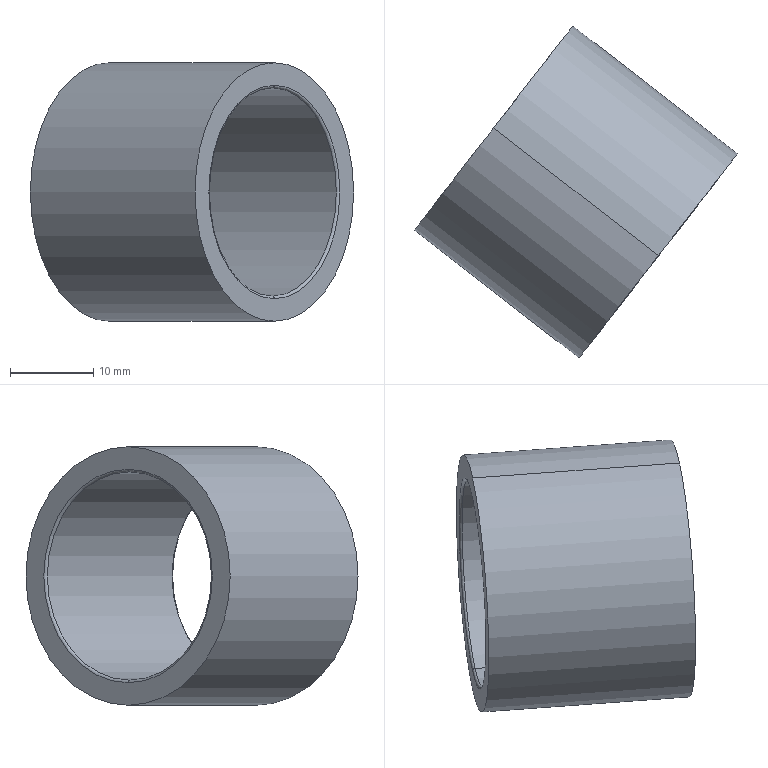Component | SolidWorks | MISUMI_BSSRK3210-800-F34-P20-1_COLLAR_MISUMI_BSSRK3210-800-F34-P20-1 | 1 solid | 10 faces | box 38.76 x 39.82 x 31 mm | volume 6594 mm3 | cylinder 4 | torus 4 | plane 2 | commonest cylinder face diameters 31 x2 25 x2
build123d program:
from build123d import *


with BuildPart() as part:
    # Sketch1 → Revolve1 (revolve)
    with BuildSketch(Plane.XY, mode=Mode.PRIVATE) as revolve1_sk:
        with BuildLine():
            Line((0.3, 12.5), (24.7, 12.5))
            ThreePointArc((24.7, 12.5), (24.912, 12.588), (25, 12.8))
            Line((25, 12.8), (25, 15.5))
            Line((25, 15.5), (0, 15.5))
            Line((0, 15.5), (0, 12.8))
            ThreePointArc((0, 12.8), (0.08787, 12.588), (0.3, 12.5))
        make_face()
    revolve(revolve1_sk.sketch.rotate(Axis((0, 0, 0), (1, 0, 0)), 90), axis=Axis((0, 0, 0), (1, 0, 0)))


solid = part.part

# Placed as in the assembly
solid = solid.moved(Location((-94.863, 818.28, 276.411), (-65.606, 35.259, -14.67)))
STEP:
#1=COLOUR_RGB('',0.7922,0.8196,0.9333);
#2=FILL_AREA_STYLE_COLOUR('',#1);
#3=FILL_AREA_STYLE('',(#2));
#4=SURFACE_STYLE_FILL_AREA(#3);
#5=SURFACE_SIDE_STYLE('',(#4));
#6=SURFACE_STYLE_USAGE(.BOTH.,#5);
#7=PRESENTATION_STYLE_ASSIGNMENT((#6));
#8=CARTESIAN_POINT('',(-3.735,32.216,11.493));
#9=VERTEX_POINT('',#8);
#10=CARTESIAN_POINT('',(-3.735,32.216,10.272));
#11=VERTEX_POINT('',#10);
#12=CARTESIAN_POINT('',(-3.735,32.216,10.882));
#13=DIRECTION('',(0.7899,-0.6132,-0.));
#14=DIRECTION('',(-0.,-0.,1.));
#15=AXIS2_PLACEMENT_3D('',#12,#13,#14);
#16=CIRCLE('',#15,0.6102);
#17=EDGE_CURVE('',#9,#11,#16,.T.);
#18=ORIENTED_EDGE('',*,*,#17,.T.);
#19=CARTESIAN_POINT('',(-2.957,31.612,10.272));
#20=VERTEX_POINT('',#19);
#21=CARTESIAN_POINT('',(-2.957,31.612,10.272));
#22=DIRECTION('',(0.7899,-0.6132,-0.));
#23=VECTOR('',#22,39.37);
#24=LINE('',#21,#23);
#25=EDGE_CURVE('',#11,#20,#24,.T.);
#26=ORIENTED_EDGE('',*,*,#25,.T.);
#27=CARTESIAN_POINT('',(-2.957,31.612,11.493));
#28=VERTEX_POINT('',#27);
#29=CARTESIAN_POINT('',(-2.957,31.612,10.882));
#30=DIRECTION('',(0.7899,-0.6132,-0.));
#31=DIRECTION('',(-0.,-0.,1.));
#32=AXIS2_PLACEMENT_3D('',#29,#30,#31);
#33=CIRCLE('',#32,0.6102);
#34=EDGE_CURVE('',#28,#20,#33,.T.);
#35=ORIENTED_EDGE('',*,*,#34,.F.);
#36=CARTESIAN_POINT('',(-2.957,31.612,11.493));
#37=DIRECTION('',(0.7899,-0.6132,-0.));
#38=VECTOR('',#37,39.37);
#39=LINE('',#36,#38);
#40=EDGE_CURVE('',#9,#28,#39,.T.);
#41=ORIENTED_EDGE('',*,*,#40,.F.);
#42=EDGE_LOOP('',(#18,#26,#35,#41));
#43=FACE_OUTER_BOUND('',#42,.T.);
#44=CARTESIAN_POINT('',(-2.957,31.612,10.882));
#45=DIRECTION('',(0.7899,-0.6132,-0.));
#46=DIRECTION('',(-0.,-0.,1.));
#47=AXIS2_PLACEMENT_3D('',#44,#45,#46);
#48=CYLINDRICAL_SURFACE('',#47,0.6102);
#49=ADVANCED_FACE('',(#43),#48,.T.);
#50=CARTESIAN_POINT('',(-3.725,32.208,11.374));
#51=VERTEX_POINT('',#50);
#52=CARTESIAN_POINT('',(-3.725,32.208,10.39));
#53=VERTEX_POINT('',#52);
#54=CARTESIAN_POINT('',(-3.725,32.208,10.882));
#55=DIRECTION('',(0.7899,-0.6132,-0.));
#56=DIRECTION('',(-0.,-0.,1.));
#57=AXIS2_PLACEMENT_3D('',#54,#55,#56);
#58=CIRCLE('',#57,0.4921);
#59=EDGE_CURVE('',#51,#53,#58,.T.);
#60=ORIENTED_EDGE('',*,*,#59,.T.);
#61=CARTESIAN_POINT('',(-3.735,32.216,10.378));
#62=VERTEX_POINT('',#61);
#63=CARTESIAN_POINT('',(-3.725,32.208,10.378));
#64=DIRECTION('',(-0.6132,-0.7899,-0.));
#65=DIRECTION('',(0.7899,-0.6132,0.));
#66=AXIS2_PLACEMENT_3D('',#63,#64,#65);
#67=CIRCLE('',#66,0.01181);
#68=EDGE_CURVE('',#53,#62,#67,.T.);
#69=ORIENTED_EDGE('',*,*,#68,.T.);
#70=CARTESIAN_POINT('',(-3.735,32.216,11.386));
#71=VERTEX_POINT('',#70);
#72=CARTESIAN_POINT('',(-3.735,32.216,10.882));
#73=DIRECTION('',(0.7899,-0.6132,-0.));
#74=DIRECTION('',(-0.,-0.,1.));
#75=AXIS2_PLACEMENT_3D('',#72,#73,#74);
#76=CIRCLE('',#75,0.5039);
#77=EDGE_CURVE('',#71,#62,#76,.T.);
#78=ORIENTED_EDGE('',*,*,#77,.F.);
#79=CARTESIAN_POINT('',(-3.725,32.208,11.386));
#80=DIRECTION('',(0.6132,0.7899,0.));
#81=DIRECTION('',(-0.7899,0.6132,0.));
#82=AXIS2_PLACEMENT_3D('',#79,#80,#81);
#83=CIRCLE('',#82,0.01181);
#84=EDGE_CURVE('',#51,#71,#83,.T.);
#85=ORIENTED_EDGE('',*,*,#84,.F.);
#86=EDGE_LOOP('',(#60,#69,#78,#85));
#87=FACE_OUTER_BOUND('',#86,.T.);
#88=CARTESIAN_POINT('',(-3.725,32.208,10.882));
#89=DIRECTION('',(0.7899,-0.6132,-0.));
#90=DIRECTION('',(-0.,-0.,1.));
#91=AXIS2_PLACEMENT_3D('',#88,#89,#90);
#92=TOROIDAL_SURFACE('',#91,0.5039,0.01181);
#93=ADVANCED_FACE('',(#87),#92,.T.);
#94=CARTESIAN_POINT('',(-3.725,32.208,10.882));
#95=DIRECTION('',(0.7899,-0.6132,-0.));
#96=DIRECTION('',(-0.,-0.,1.));
#97=AXIS2_PLACEMENT_3D('',#94,#95,#96);
#98=CIRCLE('',#97,0.4921);
#99=EDGE_CURVE('',#53,#51,#98,.T.);
#100=ORIENTED_EDGE('',*,*,#99,.F.);
#101=CARTESIAN_POINT('',(-2.967,31.619,10.39));
#102=VERTEX_POINT('',#101);
#103=CARTESIAN_POINT('',(-2.957,31.612,10.39));
#104=DIRECTION('',(0.7899,-0.6132,-0.));
#105=VECTOR('',#104,39.37);
#106=LINE('',#103,#105);
#107=EDGE_CURVE('',#53,#102,#106,.T.);
#108=ORIENTED_EDGE('',*,*,#107,.T.);
#109=CARTESIAN_POINT('',(-2.967,31.619,11.374));
#110=VERTEX_POINT('',#109);
#111=CARTESIAN_POINT('',(-2.967,31.619,10.882));
#112=DIRECTION('',(0.7899,-0.6132,-0.));
#113=DIRECTION('',(-0.,-0.,1.));
#114=AXIS2_PLACEMENT_3D('',#111,#112,#113);
#115=CIRCLE('',#114,0.4921);
#116=EDGE_CURVE('',#102,#110,#115,.T.);
#117=ORIENTED_EDGE('',*,*,#116,.T.);
#118=CARTESIAN_POINT('',(-2.957,31.612,11.374));
#119=DIRECTION('',(0.7899,-0.6132,-0.));
#120=VECTOR('',#119,39.37);
#121=LINE('',#118,#120);
#122=EDGE_CURVE('',#51,#110,#121,.T.);
#123=ORIENTED_EDGE('',*,*,#122,.F.);
#124=EDGE_LOOP('',(#100,#108,#117,#123));
#125=FACE_OUTER_BOUND('',#124,.T.);
#126=CARTESIAN_POINT('',(-2.957,31.612,10.882));
#127=DIRECTION('',(0.7899,-0.6132,-0.));
#128=DIRECTION('',(-0.,-0.,1.));
#129=AXIS2_PLACEMENT_3D('',#126,#127,#128);
#130=CYLINDRICAL_SURFACE('',#129,0.4921);
#131=ADVANCED_FACE('',(#125),#130,.F.);
#132=CARTESIAN_POINT('',(-2.957,31.612,11.386));
#133=VERTEX_POINT('',#132);
#134=CARTESIAN_POINT('',(-2.957,31.612,10.378));
#135=VERTEX_POINT('',#134);
#136=CARTESIAN_POINT('',(-2.957,31.612,10.882));
#137=DIRECTION('',(0.7899,-0.6132,-0.));
#138=DIRECTION('',(-0.,-0.,1.));
#139=AXIS2_PLACEMENT_3D('',#136,#137,#138);
#140=CIRCLE('',#139,0.5039);
#141=EDGE_CURVE('',#133,#135,#140,.T.);
#142=ORIENTED_EDGE('',*,*,#141,.T.);
#143=CARTESIAN_POINT('',(-2.967,31.619,10.378));
#144=DIRECTION('',(-0.6132,-0.7899,-0.));
#145=DIRECTION('',(0.7899,-0.6132,0.));
#146=AXIS2_PLACEMENT_3D('',#143,#144,#145);
#147=CIRCLE('',#146,0.01181);
#148=EDGE_CURVE('',#135,#102,#147,.T.);
#149=ORIENTED_EDGE('',*,*,#148,.T.);
#150=CARTESIAN_POINT('',(-2.967,31.619,10.882));
#151=DIRECTION('',(0.7899,-0.6132,-0.));
#152=DIRECTION('',(-0.,-0.,1.));
#153=AXIS2_PLACEMENT_3D('',#150,#151,#152);
#154=CIRCLE('',#153,0.4921);
#155=EDGE_CURVE('',#110,#102,#154,.T.);
#156=ORIENTED_EDGE('',*,*,#155,.F.);
#157=CARTESIAN_POINT('',(-2.967,31.619,11.386));
#158=DIRECTION('',(0.6132,0.7899,0.));
#159=DIRECTION('',(-0.7899,0.6132,0.));
#160=AXIS2_PLACEMENT_3D('',#157,#158,#159);
#161=CIRCLE('',#160,0.01181);
#162=EDGE_CURVE('',#133,#110,#161,.T.);
#163=ORIENTED_EDGE('',*,*,#162,.F.);
#164=EDGE_LOOP('',(#142,#149,#156,#163));
#165=FACE_OUTER_BOUND('',#164,.T.);
#166=CARTESIAN_POINT('',(-2.967,31.619,10.882));
#167=DIRECTION('',(0.7899,-0.6132,-0.));
#168=DIRECTION('',(-0.,-0.,1.));
#169=AXIS2_PLACEMENT_3D('',#166,#167,#168);
#170=TOROIDAL_SURFACE('',#169,0.5039,0.01181);
#171=ADVANCED_FACE('',(#165),#170,.T.);
#172=ORIENTED_EDGE('',*,*,#148,.F.);
#173=CARTESIAN_POINT('',(-2.957,31.612,10.882));
#174=DIRECTION('',(0.7899,-0.6132,-0.));
#175=DIRECTION('',(-0.,-0.,1.));
#176=AXIS2_PLACEMENT_3D('',#173,#174,#175);
#177=CIRCLE('',#176,0.5039);
#178=EDGE_CURVE('',#135,#133,#177,.T.);
#179=ORIENTED_EDGE('',*,*,#178,.T.);
#180=ORIENTED_EDGE('',*,*,#162,.T.);
#181=ORIENTED_EDGE('',*,*,#116,.F.);
#182=EDGE_LOOP('',(#172,#179,#180,#181));
#183=FACE_OUTER_BOUND('',#182,.T.);
#184=CARTESIAN_POINT('',(-2.967,31.619,10.882));
#185=DIRECTION('',(0.7899,-0.6132,-0.));
#186=DIRECTION('',(-0.,-0.,1.));
#187=AXIS2_PLACEMENT_3D('',#184,#185,#186);
#188=TOROIDAL_SURFACE('',#187,0.5039,0.01181);
#189=ADVANCED_FACE('',(#183),#188,.T.);
#190=ORIENTED_EDGE('',*,*,#107,.F.);
#191=ORIENTED_EDGE('',*,*,#59,.F.);
#192=ORIENTED_EDGE('',*,*,#122,.T.);
#193=ORIENTED_EDGE('',*,*,#155,.T.);
#194=EDGE_LOOP('',(#190,#191,#192,#193));
#195=FACE_OUTER_BOUND('',#194,.T.);
#196=CARTESIAN_POINT('',(-2.957,31.612,10.882));
#197=DIRECTION('',(0.7899,-0.6132,-0.));
#198=DIRECTION('',(-0.,-0.,1.));
#199=AXIS2_PLACEMENT_3D('',#196,#197,#198);
#200=CYLINDRICAL_SURFACE('',#199,0.4921);
#201=ADVANCED_FACE('',(#195),#200,.F.);
#202=ORIENTED_EDGE('',*,*,#68,.F.);
#203=ORIENTED_EDGE('',*,*,#99,.T.);
#204=ORIENTED_EDGE('',*,*,#84,.T.);
#205=CARTESIAN_POINT('',(-3.735,32.216,10.882));
#206=DIRECTION('',(0.7899,-0.6132,-0.));
#207=DIRECTION('',(-0.,-0.,1.));
#208=AXIS2_PLACEMENT_3D('',#205,#206,#207);
#209=CIRCLE('',#208,0.5039);
#210=EDGE_CURVE('',#62,#71,#209,.T.);
#211=ORIENTED_EDGE('',*,*,#210,.F.);
#212=EDGE_LOOP('',(#202,#203,#204,#211));
#213=FACE_OUTER_BOUND('',#212,.T.);
#214=CARTESIAN_POINT('',(-3.725,32.208,10.882));
#215=DIRECTION('',(0.7899,-0.6132,-0.));
#216=DIRECTION('',(-0.,-0.,1.));
#217=AXIS2_PLACEMENT_3D('',#214,#215,#216);
#218=TOROIDAL_SURFACE('',#217,0.5039,0.01181);
#219=ADVANCED_FACE('',(#213),#218,.T.);
#220=ORIENTED_EDGE('',*,*,#17,.F.);
#221=CARTESIAN_POINT('',(-3.735,32.216,10.882));
#222=DIRECTION('',(0.7899,-0.6132,-0.));
#223=DIRECTION('',(-0.,-0.,1.));
#224=AXIS2_PLACEMENT_3D('',#221,#222,#223);
#225=CIRCLE('',#224,0.6102);
#226=EDGE_CURVE('',#11,#9,#225,.T.);
#227=ORIENTED_EDGE('',*,*,#226,.F.);
#228=EDGE_LOOP('',(#220,#227));
#229=FACE_OUTER_BOUND('',#228,.T.);
#230=ORIENTED_EDGE('',*,*,#77,.T.);
#231=ORIENTED_EDGE('',*,*,#210,.T.);
#232=EDGE_LOOP('',(#230,#231));
#233=FACE_BOUND('',#232,.T.);
#234=CARTESIAN_POINT('',(-4.044,31.818,10.882));
#235=DIRECTION('',(0.7899,-0.6132,-0.));
#236=DIRECTION('',(-0.,-0.,1.));
#237=AXIS2_PLACEMENT_3D('',#234,#235,#236);
#238=PLANE('',#237);
#239=ADVANCED_FACE('',(#229,#233),#238,.F.);
#240=ORIENTED_EDGE('',*,*,#25,.F.);
#241=ORIENTED_EDGE('',*,*,#226,.T.);
#242=ORIENTED_EDGE('',*,*,#40,.T.);
#243=CARTESIAN_POINT('',(-2.957,31.612,10.882));
#244=DIRECTION('',(0.7899,-0.6132,-0.));
#245=DIRECTION('',(-0.,-0.,1.));
#246=AXIS2_PLACEMENT_3D('',#243,#244,#245);
#247=CIRCLE('',#246,0.6102);
#248=EDGE_CURVE('',#20,#28,#247,.T.);
#249=ORIENTED_EDGE('',*,*,#248,.F.);
#250=EDGE_LOOP('',(#240,#241,#242,#249));
#251=FACE_OUTER_BOUND('',#250,.T.);
#252=CARTESIAN_POINT('',(-2.957,31.612,10.882));
#253=DIRECTION('',(0.7899,-0.6132,-0.));
#254=DIRECTION('',(-0.,-0.,1.));
#255=AXIS2_PLACEMENT_3D('',#252,#253,#254);
#256=CYLINDRICAL_SURFACE('',#255,0.6102);
#257=ADVANCED_FACE('',(#251),#256,.T.);
#258=ORIENTED_EDGE('',*,*,#141,.F.);
#259=ORIENTED_EDGE('',*,*,#178,.F.);
#260=EDGE_LOOP('',(#258,#259));
#261=FACE_BOUND('',#260,.T.);
#262=ORIENTED_EDGE('',*,*,#34,.T.);
#263=ORIENTED_EDGE('',*,*,#248,.T.);
#264=EDGE_LOOP('',(#262,#263));
#265=FACE_OUTER_BOUND('',#264,.T.);
#266=CARTESIAN_POINT('',(-3.331,31.13,10.882));
#267=DIRECTION('',(-0.7899,0.6132,0.));
#268=DIRECTION('',(0.,0.,-1.));
#269=AXIS2_PLACEMENT_3D('',#266,#267,#268);
#270=PLANE('',#269);
#271=ADVANCED_FACE('',(#261,#265),#270,.F.);
#272=CLOSED_SHELL('',(#49,#93,#131,#171,#189,#201,#219,#239,#257,#271));
#273=MANIFOLD_SOLID_BREP('',#272);
#274=STYLED_ITEM('',(#7),#273);
#275=(LENGTH_UNIT()NAMED_UNIT(*)SI_UNIT($,.METRE.));
#276=LENGTH_MEASURE_WITH_UNIT(LENGTH_MEASURE(0.0254),#275);
#277=DIMENSIONAL_EXPONENTS(1.,0.,0.,0.,0.,0.,0.);
#278=(CONVERSION_BASED_UNIT('',#276)LENGTH_UNIT()NAMED_UNIT(#277));
#279=UNCERTAINTY_MEASURE_WITH_UNIT(LENGTH_MEASURE(0.00001),#278,'','');
#280=(NAMED_UNIT(*)PLANE_ANGLE_UNIT()SI_UNIT($,.RADIAN.));
#281=(NAMED_UNIT(*)SI_UNIT($,.STERADIAN.)SOLID_ANGLE_UNIT());
#282=(GEOMETRIC_REPRESENTATION_CONTEXT(3)GLOBAL_UNCERTAINTY_ASSIGNED_CONTEXT((#279))GLOBAL_UNIT_ASSIGNED_CONTEXT((#278,#280,#281))REPRESENTATION_CONTEXT('',''));
#283=MECHANICAL_DESIGN_GEOMETRIC_PRESENTATION_REPRESENTATION('',(#274),#282);
#284=PRESENTATION_LAYER_ASSIGNMENT('','',(#274));
#285=CARTESIAN_POINT('',(0.,0.,0.));
#286=DIRECTION('',(0.,0.,1.));
#287=DIRECTION('',(1.,0.,0.));
#288=AXIS2_PLACEMENT_3D('',#285,#286,#287);
#289=(LENGTH_UNIT()NAMED_UNIT(*)SI_UNIT($,.METRE.));
#290=LENGTH_MEASURE_WITH_UNIT(LENGTH_MEASURE(0.0254),#289);
#291=DIMENSIONAL_EXPONENTS(1.,0.,0.,0.,0.,0.,0.);
#292=(CONVERSION_BASED_UNIT('',#290)LENGTH_UNIT()NAMED_UNIT(#291));
#293=UNCERTAINTY_MEASURE_WITH_UNIT(LENGTH_MEASURE(0.00001),#292,'','');
#294=(NAMED_UNIT(*)PLANE_ANGLE_UNIT()SI_UNIT($,.RADIAN.));
#295=(NAMED_UNIT(*)SI_UNIT($,.STERADIAN.)SOLID_ANGLE_UNIT());
#296=(GEOMETRIC_REPRESENTATION_CONTEXT(3)GLOBAL_UNCERTAINTY_ASSIGNED_CONTEXT((#293))GLOBAL_UNIT_ASSIGNED_CONTEXT((#292,#294,#295))REPRESENTATION_CONTEXT('',''));
#297=ADVANCED_BREP_SHAPE_REPRESENTATION('',(#273,#288),#296);